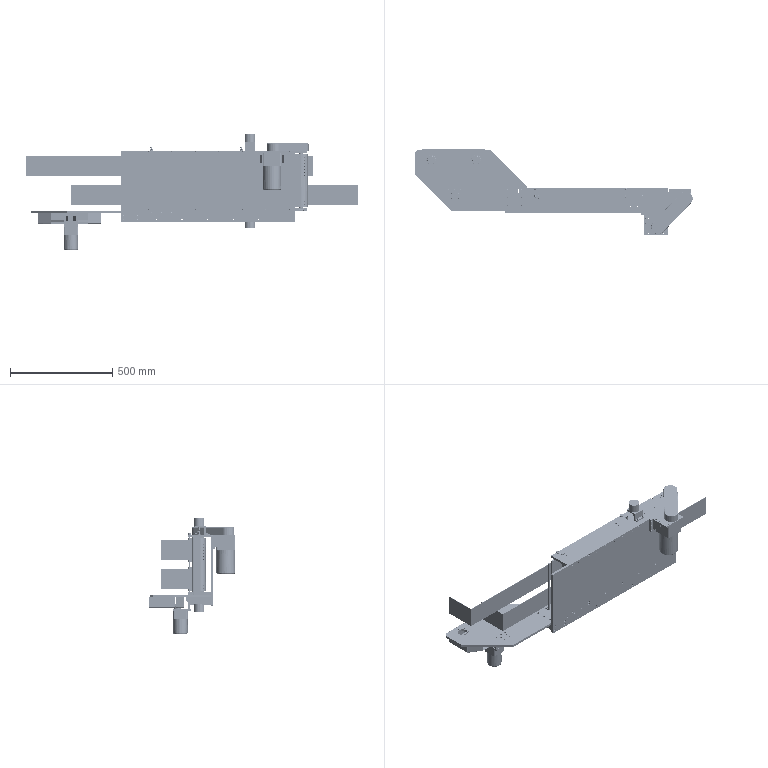Assembly | SolidWorks | mm | 75 component files | 75 solids | 4321 faces | box 1622 x 419.25 x 568 mm | volume 14757851 mm3 | cylinder 2735 | plane 960 | cone 372 | spline 244 | torus 10 | commonest cylinder face diameters 3 x1344 5 x136 4.2 x118 8 x106 5.08 x100 5.5 x93 11 x88 6.6 x88
Bill of materials:
LD101-02-35B15-d12 | 2 |  | Toothed sprocket-like disc with an integral cylindrical hub on one side and a keyed central bore; one radial hole through the hub wall.
LD101-02-35B15-d16 | 2 |  | Toothed sprocket-like disc with a tall cylindrical hub, a keyed bore and a radial hole in the hub.
LD101-02-5IK60Q1-C-5GN180K | 1 | SUS304 | Housing-like body: a square block with rounded corners and four corner holes, sitting on a cylindrical body, with a small off-centre shaft sticking out from a circular boss.
LD101-02-B6902zz(D15xD28x7)-2 | 4 | 60Si2Mn | Plain annular ring with flat faces and a large central bore; one face has two concentric recessed rings.
LD101-02-Chain35B-2 | 1 | 45 | Thin, closed, stadium-shaped (obround) band of constant width, rectangular in cross-section.
LD101-02-HexagonScrew-M6-2 | 4 |  | Short socket-head-cap-screw-like part: a cylindrical head with a hex socket on a plain cylindrical shank with a chamfered end.
LD101-02-HexagonScrew-M8X40-2 | 1 |  | Long socket-head-cap-screw-like part: a cylindrical head with a hex socket on a long plain cylindrical shank with a chamfered end.
LD101-02-Product-Q1-2-3 | 2 | POM (White) | Very thin L-shaped sheet or surface body: one long flat wall joined at a right angle to one short flat wall.
LD101-02-35B15-d10 | 1 |  | Toothed sprocket-like disc with an integral cylindrical hub, a small keyed bore and a radial hole in the hub.
LD101-02-3IK15Q1-C-3GN10K | 1 | SUS304 | Housing-like body: a square block with rounded corners and four corner holes over a cylindrical body, with a short plain off-centre shaft coming out of a circular boss.
LD101-02-Chain35B | 1 | 45 | Thin, closed band with a rounded-triangle outline: one long straight side and two converging sides, joined by rounded corners.
LD101-02--Q1108-1 | 1 | AL6061 | Flat rectangular plate with one large round through-hole near one end and seven smaller through-holes.
LD101-02--Q1109-1 | 1 | AL6061 | Thick rectangular plate/block with four holes through the large face and three holes drilled into one long narrow edge.
LD101-02--Q1110-1 | 2 | AL6061 | Solid block with a five-sided profile: a rectangle with one lower corner cut off by a long diagonal edge. Two holes are drilled into the flat top face.
LD101-02--Q1001-Q1-2 | 1 | AL6061 | Thin rectangular plate with six small holes in two columns of three, near the short ends. Its edges are beveled.
LD101-02--Q1004-Q1-2 | 2 | 45 | Long, slender cylinder with a bore along its axis, open at at least one end (tube or bored rod).
LD101-02--Q1005-Q1-2 | 2 | AL6061 | Long rectangular bar with two holes drilled into one end face.
LD101-02--Q1006-Q1-2 | 1 | 45 | Thin rectangular plate with fourteen parallel slots in two groups of seven, separated by a solid band. It has four corner holes, small V-notches at mid-height on the side edges, and beveled edges.
LD101-02--Q1011-Q1-2 | 8 | 45 | Roughly square, block-like solid with one large round through hole placed off-center. Two adjacent corners are chamfered.
LD101-02--Q1012-Q1-2 | 1 | AL6061 | Thin flat plate with an irregular outline: a long diagonal edge, a step down to a narrower rectangular extension, and a U-shaped slot open to an edge. It has two large round holes, each ringed by six small holes, plus many small holes and a short slot.
LD101-02--Q1014-Q1-2 | 1 | AL6061 | Thin, plain rectangular plate with three small holes drilled into one long edge.
LD101-02--Q1016-Q1-2 | 1 | 45 | Turned (rotationally symmetric) part: two large cylinder sections of equal diameter separated by a narrow groove, with stepped shaft ends of smaller diameter at both ends.
LD101-02--Q1017-Q1-2 | 1 | POM (White) | Thin-walled, open-ended tube with an obround (stadium-shaped) cross-section, perforated with a regular grid of small round holes in two bands separated by a solid band.
LD101-02--Q1020-Q1-2 | 1 | 45 | Long, slender, solid cylindrical rod with plain flat ends.
LD101-02--Q1024-Q1-2 | 1 | 45 | Solid of revolution: a long cylindrical body split by a narrow, shallow circumferential groove near mid-length, with small stepped shaft journals sticking out from both end faces.
LD101-02--Q1025-Q1-2 | 1 | 45 | Flat L-shaped (also readable as T-shaped) plate with one large round through hole in the main body, a chamfered corner, a long rounded-end slot running through the length of one arm, and small holes drilled into the side edges.
LD101-02--Q1026-Q1-2 | 1 | 45 | Flat L-shaped (also readable as T-shaped) plate, the same outline as unnamed part, but the large hole is stepped (counterbored) and one edge hole is larger. It also has a long rounded-end slot in one arm and chamfered corners.
LD101-02--Q1030-Q1-2 | 1 | AL6061 | Thin, large rectangular plate with slightly rounded corners and many small through holes, mostly in rows near the two long edges, plus a cluster of holes near one end.
LD101-02--Q1033-Q1-2 | 2 | AL6061 | Slender rectangular bar with two blind holes drilled into one end face. No other features are visible on the long faces.
LD101-02--Q1036-Q1-2 | 2 | AL6061 | Block with a stepped (L-shaped) cross-section: a thicker top flange overhangs a deeper web along its full length. Two round holes pass through the top flange.
LD101-02--Q1037-Q1-2 | 2 | AL6061 | Long rectangular bar whose height tapers along most of its length: one edge slopes from a full-height end to a shallower end. Three holes are in the top face and two holes are in the full-height end face.
LD101-02--Q1042-Q1-2 | 1 | AL6061 | Rectangular flat plate with one large off-center round through hole and eight smaller through holes near the perimeter, in two sizes.
LD101-02--Q1043-Q1-2 | 1 | AL6061 | Thick rectangular plate with 13 round through holes: three larger holes along each short edge, two medium holes inboard at each end, and three small holes in a row along one long edge.
LD101-02--Q1051-Q1-2 | 1 | AL6061 | Long, narrow flat plate with a stepped reduced-width end, two small U-shaped notches on one long edge, scattered small holes, one larger round hole, and a row of small holes along one long edge face.
LD101-02--Q1057-Q1-2 | 2 | AL6061 | Thick, nearly square plate with two chamfered corners on one edge, a large circular through bore, and five smaller round through holes around it.
LD101-02--Q1068-Q1-2 | 1 | AL6061 | Long, narrow flat plate with the same outline as unnamed part (stepped end, two edge notches, edge-face holes). It has extra small holes near one end and a second larger round hole, giving two larger through holes in total.
LD101-02--Q1069-Q1-2 | 2 | Nylon1010 | Thin flat rectangular plate or strip, long and narrow, with no visible holes or cutouts.
LD101-02--Q1070-Q1-2 | 2 | AL6061 | Thick plate-like block with a gusset-like profile: a short vertical edge at one side, then a long 45-degree-looking diagonal cut down to the opposite side. Two holes are drilled into one long flat narrow face.
LD101-02--Q1071-Q1-2 | 1 | SUS304 | Flat bar with a rounded-end (obround) outline, constant thickness and small edge rounds or chamfers. The shape resembles a rounded-end key.
LD101-02--Q1072-Q1-2 | 1 | SUS304 | Sheet-metal tray or cover: a flat base with an angled cut at each front corner and a U-shaped slot with a rounded end cut in from the front edge. Upturned flanges run along the back and sides, and partial flanges sit at the front. The back flange is taller and has four evenly spaced holes in a row.
LD101-02--Q1107-2 | 4 | 45 | Short thick-walled cylindrical ring or collar with a central through bore, chamfered outer edges and radial holes through the outer wall.
LD101-02-RotaryEncoder-0002-2 | 2 | AL6061 | Stepped cylindrical body: a large main cylinder, a smaller coaxial pilot boss on top and a slender cylindrical shaft sticking up from the center. The top face has three small holes spaced around the boss. The bottom face has a small circular feature at the center and three small recesses spaced around it.
LD101-02-WFSP8-0.8-10-2 | 4 |  | Shape like an extension spring: the coil is shown as a solid hollow cylindrical tube, with a round wire loop or hook at each end, and the two loops are turned relative to each other.
Mates:
1. coincident | LD101-02--Q1051-Q1-2-1 face at (-400.29, -129.897, 281.257) dir (0, 1, 0) | LD101-02--Q1068-Q1-2-2 face at (-400.29, -129.897, -0.7433) dir (0, 1, 0)
2. coincident | LD101-02--Q1051-Q1-2-1 face at (-400.29, -129.897, 281.257) dir (-1, 0, 0) | LD101-02--Q1068-Q1-2-2 face at (-400.29, -129.897, -0.7433) dir (-1, 0, 0)
3. coincident | LD101-02--Q1001-Q1-2-1 face at (-420.29, -148.897, 11.257) dir (0, 0, -1) | LD101-02--Q1068-Q1-2-2 face at (-30.29, -184.897, 11.257) dir (0, 0, 1)
4. distance | LD101-02--Q1001-Q1-2-1 face at (-420.29, -148.897, 281.257) dir (-1, 0, 0) | LD101-02--Q1068-Q1-2-2 face at (-400.29, -129.897, -0.7433) dir (-1, 0, 0)
5. coincident | LD101-02--Q1001-Q1-2-1 face at (-420.29, -148.897, 281.257) dir (0, 0, 1) | LD101-02--Q1051-Q1-2-1 face at (-30.29, -184.897, 281.257) dir (0, 0, -1)
6. distance | LD101-02--Q1001-Q1-2-1 face at (-160.29, -148.897, 146.257) dir (0, 1, 0) | LD101-02--Q1068-Q1-2-2 face at (-400.29, -129.897, -0.7433) dir (0, 1, 0)
7. concentric | LD101-02--Q1004-Q1-2-1 face at (-360.29, -135.897, 303.757) dir (0, 0, -1) r 4 | LD101-02--Q1011-Q1-2-1 face at (-360.29, -135.897, 155.257) dir (0, 0, 1) r 4
8. width | LD101-02--Q1004-Q1-2-1 face at (-360.29, -135.897, 303.757) dir (0, 0, 1) | LD101-02--Q1004-Q1-2-1 face at (-360.29, -135.897, -11.243) dir (0, 0, -1) | LD101-02--Q1068-Q1-2-2 face at (-30.29, -184.897, -0.7433) dir (0, 0, -1) | LD101-02--Q1051-Q1-2-1 face at (-30.29, -184.897, 293.257) dir (0, 0, 1)
9. concentric | LD101-02--Q1004-Q1-2-1 face at (-360.29, -135.897, 303.757) dir (0, 0, -1) r 4 | LD101-02--Q1011-Q1-2-2 face at (-360.29, -135.897, 125.257) dir (0, 0, 1) r 4
10. concentric | LD101-02--Q1051-Q1-2-1 face at (-360.29, -135.897, 281.257) dir (0, 0, 1) r 4.1 | LD101-02--Q1004-Q1-2-1 face at (-360.29, -135.897, 303.757) dir (0, 0, -1) r 4
11. coincident | LD101-02--Q1011-Q1-2-1 face at (-370.29, -129.897, 167.257) dir (0, 1, 0) | LD101-02--Q1011-Q1-2-2 face at (-370.29, -129.897, 137.257) dir (0, 1, 0)
12. concentric | LD101-02--Q1004-Q1-2-2 face at (79.71, -135.897, -11.243) dir (0, 0, 1) r 4 | LD101-02--Q1011-Q1-2-3 face at (79.71, -135.897, 139.257) dir (0, 0, -1) r 4
13. concentric | LD101-02--Q1004-Q1-2-2 face at (79.71, -135.897, -11.243) dir (0, 0, 1) r 4 | LD101-02--Q1011-Q1-2-4 face at (79.71, -135.897, 169.257) dir (0, 0, -1) r 4
14. concentric | LD101-02--Q1051-Q1-2-1 face at (79.71, -135.897, 281.257) dir (0, 0, 1) r 4.1 | LD101-02--Q1004-Q1-2-2 face at (79.71, -135.897, -11.243) dir (0, 0, 1) r 4
15. coincident | LD101-02--Q1004-Q1-2-1 face at (-360.29, -135.897, 303.757) dir (0, 0, 1) | LD101-02--Q1004-Q1-2-2 face at (79.71, -135.897, 303.757) dir (0, 0, 1)
16. coincident | LD101-02--Q1011-Q1-2-1 face at (-360.29, -139.397, 167.257) dir (0, 0, 1) | LD101-02--Q1011-Q1-2-4 face at (79.71, -139.397, 167.257) dir (0, 0, 1)
17. coincident | LD101-02--Q1011-Q1-2-2 face at (-360.29, -139.397, 137.257) dir (0, 0, 1) | LD101-02--Q1011-Q1-2-3 face at (79.71, -139.397, 137.257) dir (0, 0, 1)
18. coincident | LD101-02--Q1011-Q1-2-3 face at (89.71, -129.897, 127.257) dir (0, 1, 0) | LD101-02--Q1011-Q1-2-4 face at (89.71, -129.897, 157.257) dir (0, 1, 0)
19. concentric | LD101-02-WFSP8-0.8-10-2-1 sketch segment at (-360.29, -175.897, 299.257) dir (0, 0, 1) r 3.2 | LD101-02-HexagonScrew-M6-2-1 face at (-360.29, -175.897, 301.563) dir (0, 0, -1) r 3
20. concentric | LD101-02-WFSP8-0.8-10-2-4 sketch segment at (79.71, -175.897, 299.257) dir (0, 0, 1) r 3.2 | LD101-02-HexagonScrew-M6-2-4 face at (79.71, -175.897, 301.563) dir (0, 0, -1) r 3
21. parallel | LD101-02--Q1051-Q1-2-1 face at (339.71, -129.897, 281.257) dir (1, 0, 0) | LD101-02-WFSP8-0.8-10-2-4 plane at (79.71, -179.097, 299.257) dir (-1, 0, 0)
22. concentric | LD101-02--Q1004-Q1-2-1 face at (-360.29, -135.897, 303.757) dir (0, 0, -1) r 4 | LD101-02--Q1107-2-1 face at (-360.29, -135.897, 299.257) dir (0, 0, -1) r 4
23. coincident | LD101-02--Q1051-Q1-2-1 face at (-30.29, -184.897, 293.257) dir (0, 0, 1) | LD101-02--Q1107-2-1 face at (-360.29, -135.897, 293.257) dir (0, 0, -1)
24. coincident | LD101-02--Q1107-2-1 face at (-360.29, -135.897, 299.257) dir (0, 0, 1) | LD101-02--Q1107-2-5 face at (79.71, -135.897, 299.257) dir (0, 0, 1)
25. concentric | LD101-02--Q1004-Q1-2-2 face at (79.71, -135.897, -11.243) dir (0, 0, 1) r 4 | LD101-02--Q1107-2-5 face at (79.71, -135.897, 299.257) dir (0, 0, -1) r 4
26. width | LD101-02--Q1051-Q1-2-1 face at (-30.29, -184.897, 281.257) dir (0, 0, -1) | LD101-02--Q1068-Q1-2-2 face at (-30.29, -184.897, 11.257) dir (0, 0, 1) | LD101-02--Q1016-Q1-2-1 face at (121.71, -181.897, 16.257) dir (0, 0, -1) | LD101-02--Q1016-Q1-2-1 face at (121.71, -181.897, 276.257) dir (0, 0, 1)
27. concentric | LD101-02--Q1016-Q1-2-1 face at (121.71, -181.897, -3.743) dir (0, 0, 1) r 7.5 | LD101-02--Q1017-Q1-2-1 face at (121.71, -181.897, 276.257) dir (0, 0, -1) r 30
28. coincident | LD101-02--Q1016-Q1-2-1 face at (121.71, -181.897, 276.257) dir (0, 0, 1) | LD101-02--Q1017-Q1-2-1 face at (121.71, -181.897, 276.257) dir (0, 0, 1)
29. concentric | LD101-02--Q1016-Q1-2-1 face at (121.71, -181.897, 296.257) dir (0, 0, -1) r 7.5 | LD101-02-B6902zz(D15xD28x7)-2-1 face at (121.71, -181.897, 289.757) dir (0, 0, 1) r 7.5
30. coincident | LD101-02--Q1016-Q1-2-1 face at (121.71, -181.897, 286.257) dir (0, 0, 1) | LD101-02-B6902zz(D15xD28x7)-2-1 face at (117.578, -174.412, 286.257) dir (0, 0, -1)
31. concentric | LD101-02--Q1016-Q1-2-1 face at (121.71, -181.897, -3.743) dir (0, 0, 1) r 7.5 | LD101-02-B6902zz(D15xD28x7)-2-2 face at (121.71, -181.897, 2.757) dir (0, 0, 1) r 14
32. coincident | LD101-02--Q1016-Q1-2-1 face at (121.71, -181.897, 6.257) dir (0, 0, -1) | LD101-02-B6902zz(D15xD28x7)-2-2 face at (121.71, -173.347, 6.257) dir (0, 0, 1)
33. concentric | LD101-02--Q1017-Q1-2-1 face at (371.71, -181.897, 276.257) dir (0, 0, -1) r 30 | LD101-02--Q1024-Q1-2-1 face at (371.71, -181.897, 291.257) dir (0, 0, -1) r 7.5
34. concentric | LD101-02--Q1024-Q1-2-1 face at (371.71, -181.897, 291.257) dir (0, 0, -1) r 7.5 | LD101-02--Q1025-Q1-2-1 face at (371.71, -181.897, 288.257) dir (0, 0, -1) r 14
35. coincident | LD101-02--Q1024-Q1-2-1 face at (371.71, -181.897, 281.257) dir (0, 0, 1) | LD101-02--Q1025-Q1-2-1 face at (346.71, -132.897, 281.257) dir (0, 0, -1)
36. concentric | LD101-02--Q1024-Q1-2-1 face at (371.71, -181.897, 316.257) dir (0, 0, 1) r 6 | LD101-02--Q1026-Q1-2-1 face at (371.71, -181.897, 4.257) dir (0, 0, 1) r 14
37. coincident | LD101-02--Q1024-Q1-2-1 face at (371.71, -181.897, 11.257) dir (0, 0, -1) | LD101-02--Q1026-Q1-2-1 face at (346.71, -132.897, 11.257) dir (0, 0, 1)
38. coincident | LD101-02--Q1017-Q1-2-1 face at (121.71, -181.897, 276.257) dir (0, 0, 1) | LD101-02--Q1024-Q1-2-1 face at (371.71, -181.897, 276.257) dir (0, 0, 1)
39. coincident | LD101-02--Q1025-Q1-2-1 face at (401.71, -132.897, 293.257) dir (0, 1, 0) | LD101-02--Q1026-Q1-2-1 face at (401.71, -132.897, 11.257) dir (0, 1, 0)
40. parallel | LD101-02--Q1051-Q1-2-1 face at (-400.29, -129.897, 281.257) dir (0, 1, 0) | LD101-02--Q1025-Q1-2-1 face at (401.71, -132.897, 293.257) dir (0, 1, 0)
41. width | LD101-02--Q1068-Q1-2-2 face at (-30.29, -184.897, 11.257) dir (0, 0, 1) | LD101-02--Q1051-Q1-2-1 face at (-30.29, -184.897, 281.257) dir (0, 0, -1) | LD101-02--Q1069-Q1-2-2 face at (-370.29, -153.897, 279.257) dir (0, 0, 1) | LD101-02--Q1069-Q1-2-2 face at (-370.29, -153.897, 13.257) dir (0, 0, -1)
42. parallel | LD101-02--Q1051-Q1-2-1 face at (-400.29, -129.897, 281.257) dir (0, 1, 0) | LD101-02--Q1011-Q1-2-1 face at (-370.29, -129.897, 167.257) dir (0, 1, 0)
43. coincident | LD101-02--Q1069-Q1-2-2 face at (-370.29, -153.897, 13.257) dir (1, 0, 0) | LD101-02--Q1011-Q1-2-2 face at (-370.29, -148.897, 137.257) dir (-1, 0, 0)
44. width | LD101-02--Q1051-Q1-2-1 face at (-30.29, -184.897, 281.257) dir (0, 0, -1) | LD101-02--Q1068-Q1-2-2 face at (-30.29, -184.897, 11.257) dir (0, 0, 1) | LD101-02--Q1069-Q1-2-3 face at (69.71, -153.897, 279.257) dir (0, 0, 1) | LD101-02--Q1069-Q1-2-3 face at (69.71, -153.897, 13.257) dir (0, 0, -1)
45. coincident | LD101-02--Q1011-Q1-2-4 face at (69.71, -148.897, 157.257) dir (-1, 0, 0) | LD101-02--Q1069-Q1-2-3 face at (69.71, -153.897, 13.257) dir (1, 0, 0)
46. parallel | LD101-02--Q1051-Q1-2-1 face at (-400.29, -129.897, 281.257) dir (0, 1, 0) | LD101-02--Q1017-Q1-2-1 face at (121.71, -148.897, 276.257) dir (0, 1, 0)
47. concentric | LD101-02-HexagonScrew-M6-2-4 face at (79.71, -175.897, 301.563) dir (0, 0, -1) r 3 | LD101-02--Q1051-Q1-2-1 face at (79.71, -175.897, 293.257) dir (0, 0, 1) r 3
48. distance | LD101-02-HexagonScrew-M6-2-4 face at (79.71, -175.897, 285.257) dir (0, 0, -1) | LD101-02--Q1051-Q1-2-1 face at (-30.29, -184.897, 293.257) dir (0, 0, 1)
49. coincident | LD101-02--Q1051-Q1-2-1 face at (-400.29, -239.897, 281.257) dir (0, -1, 0) | LD101-02--Q1030-Q1-2-1 face at (-85.29, -239.897, 118.257) dir (0, 1, 0)
50. coincident | LD101-02--Q1068-Q1-2-2 face at (-30.29, -184.897, 11.257) dir (0, 0, 1) | LD101-02--Q1014-Q1-2-1 face at (244.21, -200.897, 11.257) dir (0, 0, -1)
51. coincident | LD101-02--Q1014-Q1-2-1 face at (159.21, -196.897, 281.257) dir (0, 1, 0) | LD101-02--Q1005-Q1-2-1 face at (164.21, -196.897, 146.257) dir (0, -1, 0)
52. coincident | LD101-02--Q1068-Q1-2-2 face at (-30.29, -184.897, 11.257) dir (0, 0, 1) | LD101-02--Q1005-Q1-2-1 face at (160.21, -196.897, 11.257) dir (0, 0, -1)
53. distance | LD101-02--Q1014-Q1-2-1 face at (159.21, -204.897, 281.257) dir (-1, 0, 0) | LD101-02--Q1005-Q1-2-1 face at (160.21, -196.897, 281.257) dir (-1, 0, 0)
54. coincident | LD101-02--Q1005-Q1-2-1 face at (160.21, -196.897, 281.257) dir (0, 0, 1) | LD101-02--Q1005-Q1-2-2 face at (320.21, -196.897, 281.257) dir (0, 0, 1)
55. coincident | LD101-02--Q1005-Q1-2-1 face at (164.21, -160.897, 146.257) dir (0, 1, 0) | LD101-02--Q1005-Q1-2-2 face at (324.21, -160.897, 146.257) dir (0, 1, 0)
56. distance | LD101-02--Q1005-Q1-2-2 face at (328.21, -196.897, 281.257) dir (1, 0, 0) | LD101-02--Q1014-Q1-2-1 face at (329.21, -204.897, 281.257) dir (1, 0, 0)
57. coincident | LD101-02--Q1005-Q1-2-1 face at (164.21, -160.897, 146.257) dir (0, 1, 0) | LD101-02--Q1006-Q1-2-1 face at (154.21, -160.897, 281.257) dir (0, -1, 0)
58. coincident | LD101-02--Q1005-Q1-2-1 face at (160.21, -196.897, 281.257) dir (0, 0, 1) | LD101-02--Q1006-Q1-2-1 face at (244.21, -156.897, 281.257) dir (0, 0, 1)
59. width | LD101-02--Q1006-Q1-2-1 face at (154.21, -160.897, 281.257) dir (-1, 0, 0) | LD101-02--Q1006-Q1-2-1 face at (334.21, -160.897, 281.257) dir (1, 0, 0) | LD101-02--Q1005-Q1-2-2 face at (328.21, -196.897, 281.257) dir (1, 0, 0) | LD101-02--Q1005-Q1-2-1 face at (160.21, -196.897, 281.257) dir (-1, 0, 0)
60. coincident | LD101-02--Q1068-Q1-2-2 face at (-30.29, -184.897, -0.7433) dir (0, 0, -1) | LD101-02--Q1012-Q1-2-5 face at (-600.29, -89.897, -0.7433) dir (0, 0, 1)
61. coincident | LD101-02--Q1030-Q1-2-1 face at (-85.29, -239.897, 118.257) dir (0, 1, 0) | LD101-02--Q1012-Q1-2-5 face at (-950.29, -239.897, -12.743) dir (0, -1, 0)
62. distance | LD101-02--Q1012-Q1-2-5 face at (-250.29, 60.103, -12.743) dir (1, 0, 0) | LD101-02--Q1068-Q1-2-2 face at (-400.29, -129.897, -0.7433) dir (-1, 0, 0)
63. coincident | LD101-02--Q1051-Q1-2-1 face at (339.71, -129.897, 281.257) dir (1, 0, 0) | LD101-02--Q1030-Q1-2-1 face at (339.71, -239.897, 293.257) dir (1, 0, 0)
64. coincident | LD101-02--Q1020-Q1-2-1 face at (-440.29, -154.897, -0.7433) dir (0, 0, -1) | LD101-02--Q1012-Q1-2-5 face at (-600.29, -89.897, -0.7433) dir (0, 0, 1)
65. concentric | LD101-02--Q1026-Q1-2-1 face at (361.71, -212.897, 5.257) dir (1, 0, 0) r 4 | LD101-02-HexagonScrew-M8X40-2-2 face at (375.094, -212.897, 5.257) dir (-1, 0, 0) r 4
66. coincident | LD101-02--Q1068-Q1-2-2 face at (339.71, -129.897, -0.7433) dir (1, 0, 0) | LD101-02-HexagonScrew-M8X40-2-2 face at (339.71, -212.897, 5.257) dir (-1, 0, 0)
67. coincident | LD101-02--Q1001-Q1-2-1 face at (-160.29, -156.897, 146.257) dir (0, -1, 0) | LD101-02--Q1033-Q1-2-1 face at (-350.29, -156.897, 11.257) dir (0, 1, 0)
68. width | LD101-02--Q1051-Q1-2-1 face at (-30.29, -184.897, 281.257) dir (0, 0, -1) | LD101-02--Q1068-Q1-2-2 face at (-30.29, -184.897, 11.257) dir (0, 0, 1) | LD101-02--Q1033-Q1-2-1 face at (-350.29, -186.897, 281.257) dir (0, 0, 1) | LD101-02--Q1033-Q1-2-1 face at (-350.29, -186.897, 11.257) dir (0, 0, -1)
69. coincident | LD101-02--Q1033-Q1-2-1 face at (-350.29, -186.897, 281.257) dir (0, 0, 1) | LD101-02--Q1033-Q1-2-2 face at (9.71, -186.897, 281.257) dir (0, 0, 1)
70. coincident | LD101-02--Q1033-Q1-2-1 face at (-350.29, -186.897, 11.257) dir (0, -1, 0) | LD101-02--Q1033-Q1-2-2 face at (9.71, -186.897, 11.257) dir (0, -1, 0)
71. distance | LD101-02--Q1033-Q1-2-1 face at (-350.29, -171.897, 146.257) dir (-1, 0, 0) | LD101-02--Q1068-Q1-2-2 face at (-400.29, -129.897, -0.7433) dir (-1, 0, 0)
72. coincident | LD101-02--Q1025-Q1-2-1 face at (371.71, -181.897, 288.257) dir (0, 0, -1) | LD101-02-B6902zz(D15xD28x7)-2-3 face at (371.71, -173.347, 288.257) dir (0, 0, 1)
73. concentric | LD101-02--Q1025-Q1-2-1 face at (371.71, -181.897, 288.257) dir (0, 0, -1) r 14 | LD101-02-B6902zz(D15xD28x7)-2-3 face at (371.71, -181.897, 284.757) dir (0, 0, 1) r 7.5
74. concentric | LD101-02--Q1026-Q1-2-1 face at (371.71, -181.897, 4.257) dir (0, 0, 1) r 14 | LD101-02-B6902zz(D15xD28x7)-2-4 face at (371.71, -181.897, 7.757) dir (0, 0, 1) r 7.5
75. coincident | LD101-02--Q1026-Q1-2-1 face at (371.71, -181.897, 4.257) dir (0, 0, 1) | LD101-02-B6902zz(D15xD28x7)-2-4 face at (371.71, -173.347, 4.257) dir (0, 0, -1)
76. coincident | LD101-02--Q1030-Q1-2-1 face at (-85.29, -239.897, 118.257) dir (0, 1, 0) | LD101-02--Q1037-Q1-2-1 face at (-488.29, -239.897, -12.743) dir (0, -1, 0)
77. coincident | LD101-02--Q1012-Q1-2-5 face at (-600.29, -89.897, -12.743) dir (0, 0, -1) | LD101-02--Q1037-Q1-2-1 face at (-488.29, -119.897, -12.743) dir (0, 0, 1)
78. distance | LD101-02--Q1037-Q1-2-1 face at (-500.29, -239.897, -12.743) dir (-1, 0, 0) | LD101-02--Q1030-Q1-2-1 face at (-510.29, -239.897, 293.257) dir (-1, 0, 0)
79. concentric | LD101-02--Q1068-Q1-2-2 face at (121.71, -181.897, 6.257) dir (0, 0, -1) r 14 | LD101-02--Q1016-Q1-2-1 face at (121.71, -181.897, -18.743) dir (0, 0, 1) r 4
80. coincident | LD101-02--Q1042-Q1-2-1 face at (170.211, -261.897, 293.257) dir (0, 1, 0) | LD101-02--Q1043-Q1-2-1 face at (229.211, -261.897, 258.257) dir (0, -1, 0)
81. coincident | LD101-02--Q1036-Q1-2-1 face at (146.71, -224.897, -35.743) dir (0, 0, -1) | LD101-02--Q1057-Q1-2-1 face at (121.71, -185.897, -35.743) dir (0, 0, 1)
82. concentric | LD101-02--Q1036-Q1-2-1 face at (139.71, -210.897, -35.743) dir (0, 0, -1) r 1.65 | LD101-02--Q1057-Q1-2-1 face at (139.71, -210.897, -43.743) dir (0, 0, -1) r 4
83. concentric | LD101-02--Q1036-Q1-2-1 face at (103.71, -210.897, -35.743) dir (0, 0, -1) r 1.65 | LD101-02--Q1057-Q1-2-1 face at (103.71, -210.897, -43.743) dir (0, 0, -1) r 4
84. concentric | LD101-02-RotaryEncoder-0002-2-1 face at (121.71, -181.897, -38.743) dir (0, 0, -1) r 15 | LD101-02--Q1057-Q1-2-1 face at (121.71, -181.897, -43.743) dir (0, 0, 1) r 15.05
85. coincident | LD101-02-RotaryEncoder-0002-2-1 face at (121.71, -181.897, -43.743) dir (0, 0, 1) | LD101-02--Q1057-Q1-2-1 face at (121.71, -185.897, -43.743) dir (0, 0, -1)
86. distance | LD101-02--Q1006-Q1-2-1 face at (154.21, -152.897, 281.257) dir (0, 1, 0) | LD101-02--Q1017-Q1-2-1 face at (121.71, -151.897, 276.257) dir (0, -1, 0)
87. distance | LD101-02--Q1014-Q1-2-1 face at (329.21, -204.897, 281.257) dir (1, 0, 0) | LD101-02--Q1068-Q1-2-2 face at (339.71, -129.897, -0.7433) dir (1, 0, 0)
88. distance | LD101-02--Q1033-Q1-2-1 face at (-340.29, -171.897, 146.257) dir (1, 0, 0) | LD101-02--Q1033-Q1-2-2 face at (9.71, -171.897, 146.257) dir (-1, 0, 0)
89. coincident | LD101-02-Product-Q1-2-3-1 face at (-750.29, -146.897, 127.257) dir (0, 1, 0) | LD101-02-Product-Q1-2-3-2 face at (-970.29, -146.897, 267.257) dir (0, 1, 0)
90. concentric | LD101-02--Q1016-Q1-2-1 face at (121.71, -181.897, -18.743) dir (0, 0, 1) r 4 | LD101-02-RotaryEncoder-0002-2-1 face at (121.71, -181.897, -23.743) dir (0, 0, -1) r 4
91. coincident | LD101-02--Q1068-Q1-2-2 face at (-30.29, -184.897, -0.7433) dir (0, 0, -1) | LD101-02--Q1036-Q1-2-1 face at (146.71, -224.897, -0.7433) dir (0, 0, 1)
92. parallel | LD101-02--Q1068-Q1-2-2 face at (-400.29, -129.897, -0.7433) dir (0, 1, 0) | LD101-02--Q1057-Q1-2-1 face at (147.71, -155.897, -35.743) dir (0, 1, 0)
93. concentric | LD101-02--Q1057-Q1-2-2 face at (121.71, -181.897, 336.257) dir (0, 0, -1) r 15.05 | LD101-02-RotaryEncoder-0002-2-2 face at (121.71, -181.897, 316.257) dir (0, 0, 1) r 4
94. coincident | LD101-02--Q1057-Q1-2-2 face at (121.71, -185.897, 336.257) dir (0, 0, 1) | LD101-02-RotaryEncoder-0002-2-2 face at (121.71, -181.897, 336.257) dir (0, 0, -1)
95. concentric | LD101-02--Q1036-Q1-2-2 face at (103.71, -210.897, 328.257) dir (0, 0, 1) r 1.65 | LD101-02--Q1057-Q1-2-2 face at (103.71, -210.897, 336.257) dir (0, 0, 1) r 4
96. coincident | LD101-02--Q1036-Q1-2-2 face at (96.71, -224.897, 328.257) dir (0, 0, 1) | LD101-02--Q1057-Q1-2-2 face at (121.71, -185.897, 328.257) dir (0, 0, -1)
97. concentric | LD101-02--Q1036-Q1-2-2 face at (139.71, -210.897, 328.257) dir (0, 0, 1) r 1.65 | LD101-02--Q1057-Q1-2-2 face at (139.71, -210.897, 336.257) dir (0, 0, 1) r 2.25
98. coincident | LD101-02--Q1051-Q1-2-1 face at (-30.29, -184.897, 293.257) dir (0, 0, 1) | LD101-02--Q1036-Q1-2-2 face at (96.71, -224.897, 293.257) dir (0, 0, -1)
99. concentric | LD101-02--Q1016-Q1-2-1 face at (121.71, -181.897, 296.257) dir (0, 0, -1) r 7.5 | LD101-02-RotaryEncoder-0002-2-2 face at (121.71, -181.897, 316.257) dir (0, 0, 1) r 4
100. parallel | LD101-02--Q1051-Q1-2-1 face at (-400.29, -129.897, 281.257) dir (0, 1, 0) | LD101-02--Q1057-Q1-2-2 face at (95.71, -155.897, 328.257) dir (0, 1, 0)
101. coincident | LD101-02-35B15-d16-1 face at (-650.227, 16.103, -52.743) dir (0, 0, -1) | LD101-02-35B15-d16-2 face at (-870.227, 16.103, -52.743) dir (0, 0, -1)
102. coincident | LD101-02--Q1012-Q1-2-5 face at (-600.29, -89.897, -12.743) dir (0, 0, -1) | LD101-02--Q1000-Q16-1.SLDQ1SM-1/LD101-02--Q1109-1-2 face at (-718.29, -139.897, -12.743) dir (0, 0, 1)
103. distance | LD101-02--Q1000-Q16-1.SLDQ1SM-1/LD101-02--Q1109-1-2 face at (-788.29, -139.897, -12.743) dir (-1, 0, 0) | LD101-02--Q1012-Q1-2-5 face at (-950.29, 60.103, -12.743) dir (-1, 0, 0)
104. distance | LD101-02--Q1000-Q16-1.SLDQ1SM-1/LD101-02--Q1109-1-2 face at (-753.29, -139.897, -41.743) dir (0, -1, 0) | LD101-02--Q1012-Q1-2-5 face at (-950.29, -239.897, -12.743) dir (0, -1, 0)
105. concentric | LD101-02--Q1020-Q1-2-1 face at (-440.29, -154.897, 279.257) dir (0, 0, -1) r 4 | LD101-02--Q1012-Q1-2-5 face at (-440.29, -154.897, -12.743) dir (0, 0, 1) r 2.75
106. coincident | LD101-02--Q1037-Q1-2-1 face at (-488.29, -239.897, -52.743) dir (0, 0, -1) | LD101-02--Q1037-Q1-2-2 face at (-421.29, -239.897, -52.743) dir (0, 0, -1)
107. coincident | LD101-02--Q1037-Q1-2-1 face at (-488.29, -119.897, -32.743) dir (0, 1, 0) | LD101-02--Q1037-Q1-2-2 face at (-421.29, -119.897, -32.743) dir (0, 1, 0)
108. distance | LD101-02--Q1037-Q1-2-2 face at (-433.29, -239.897, -12.743) dir (-1, 0, 0) | LD101-02--Q1030-Q1-2-1 face at (-510.29, -239.897, 293.257) dir (-1, 0, 0)
109. concentric | LD101-02--Q1004-Q1-2-1 face at (-360.29, -135.897, 303.757) dir (0, 0, -1) r 4 | LD101-02--Q1011-Q1-2-5 face at (-360.29, -135.897, 265.257) dir (0, 0, 1) r 4
110. concentric | LD101-02--Q1004-Q1-2-2 face at (79.71, -135.897, -11.243) dir (0, 0, 1) r 4 | LD101-02--Q1011-Q1-2-6 face at (79.71, -135.897, 279.257) dir (0, 0, -1) r 4
111. concentric | LD101-02--Q1004-Q1-2-2 face at (79.71, -135.897, -11.243) dir (0, 0, 1) r 4 | LD101-02--Q1011-Q1-2-7 face at (79.71, -135.897, 29.257) dir (0, 0, -1) r 4
112. coincident | LD101-02--Q1011-Q1-2-5 face at (-360.29, -139.397, 277.257) dir (0, 0, 1) | LD101-02--Q1011-Q1-2-6 face at (79.71, -139.397, 277.257) dir (0, 0, 1)
113. concentric | LD101-02--Q1004-Q1-2-1 face at (-360.29, -135.897, 303.757) dir (0, 0, -1) r 4 | LD101-02--Q1011-Q1-2-8 face at (-360.29, -135.897, 15.257) dir (0, 0, 1) r 4
114. coincident | LD101-02--Q1011-Q1-2-7 face at (79.71, -139.397, 27.257) dir (0, 0, 1) | LD101-02--Q1011-Q1-2-8 face at (-360.29, -139.397, 27.257) dir (0, 0, 1)
115. coincident | LD101-02--Q1068-Q1-2-2 face at (-400.29, -129.897, -0.7433) dir (0, 1, 0) | LD101-02--Q1011-Q1-2-8 face at (-370.29, -129.897, 27.257) dir (0, 1, 0)
116. coincident | LD101-02--Q1068-Q1-2-2 face at (-400.29, -129.897, -0.7433) dir (0, 1, 0) | LD101-02--Q1011-Q1-2-7 face at (89.71, -129.897, 17.257) dir (0, 1, 0)
117. distance | LD101-02--Q1011-Q1-2-7 face at (79.71, -139.397, 27.257) dir (0, 0, 1) | LD101-02--Q1068-Q1-2-2 face at (-30.29, -184.897, 11.257) dir (0, 0, 1)
118. distance | LD101-02--Q1011-Q1-2-3 face at (79.71, -139.397, 127.257) dir (0, 0, -1) | LD101-02--Q1011-Q1-2-7 face at (79.71, -139.397, 27.257) dir (0, 0, 1)
119. distance | LD101-02--Q1011-Q1-2-6 face at (79.71, -139.397, 267.257) dir (0, 0, -1) | LD101-02--Q1011-Q1-2-4 face at (79.71, -139.397, 167.257) dir (0, 0, 1)
120. distance | LD101-02--Q1011-Q1-2-6 face at (79.71, -139.397, 267.257) dir (0, 0, -1) | LD101-02--Q1051-Q1-2-1 face at (-30.29, -184.897, 281.257) dir (0, 0, -1)
121. coincident | LD101-02--Q1042-Q1-2-1 face at (229.211, -309.397, 283.257) dir (0, 0, -1) | LD101-02-5IK60Q1-C-5GN180K-1 face at (190.211, -350.897, 283.257) dir (0, 0, 1)
122. concentric | LD101-02--Q1042-Q1-2-1 face at (247.211, -311.897, 293.257) dir (0, 0, -1) r 17.1 | LD101-02-5IK60Q1-C-5GN180K-1 face at (247.211, -311.897, 287.257) dir (0, 0, -1) r 17
123. coincident | LD101-02--Q1042-Q1-2-1 face at (229.211, -309.397, 293.257) dir (0, 0, 1) | LD101-02--Q1043-Q1-2-1 face at (156.711, -251.897, 293.257) dir (0, 0, 1)
124. width | LD101-02--Q1042-Q1-2-1 face at (170.211, -356.897, 293.257) dir (-1, 0, 0) | LD101-02--Q1042-Q1-2-1 face at (288.211, -356.897, 293.257) dir (1, 0, 0) | LD101-02--Q1043-Q1-2-1 face at (156.711, -251.897, 293.257) dir (-1, 0, 0) | LD101-02--Q1043-Q1-2-1 face at (301.711, -251.897, 293.257) dir (1, 0, 0)
125. parallel | LD101-02--Q1042-Q1-2-1 face at (170.211, -356.897, 293.257) dir (0, -1, 0) | LD101-02-5IK60Q1-C-5GN180K-1 face at (190.211, -356.897, 216.257) dir (0, -1, 0)
126. coincident | LD101-02--Q1030-Q1-2-1 face at (-85.29, -251.897, 118.257) dir (0, -1, 0) | LD101-02--Q1043-Q1-2-1 face at (229.211, -251.897, 258.257) dir (0, 1, 0)
127. coincident | LD101-02--Q1070-Q1-2-1 face at (286.711, -261.897, 233.257) dir (0, 1, 0) | LD101-02--Q1070-Q1-2-2 face at (181.711, -261.897, 233.257) dir (0, 1, 0)
128. coincident | LD101-02--Q1070-Q1-2-1 face at (286.711, -261.897, 283.257) dir (0, 0, 1) | LD101-02--Q1070-Q1-2-2 face at (181.711, -261.897, 283.257) dir (0, 0, 1)
129. coincident | LD101-02--Q1042-Q1-2-1 face at (229.211, -309.397, 283.257) dir (0, 0, -1) | LD101-02--Q1070-Q1-2-2 face at (181.711, -261.897, 283.257) dir (0, 0, 1)
130. coincident | LD101-02--Q1043-Q1-2-1 face at (229.211, -261.897, 258.257) dir (0, -1, 0) | LD101-02--Q1070-Q1-2-2 face at (181.711, -261.897, 233.257) dir (0, 1, 0)
131. distance | LD101-02--Q1070-Q1-2-1 face at (276.711, -261.897, 283.257) dir (-1, 0, 0) | LD101-02-5IK60Q1-C-5GN180K-1 face at (274.211, -272.897, 216.257) dir (1, 0, 0)
132. distance | LD101-02--Q1070-Q1-2-2 face at (181.711, -261.897, 283.257) dir (1, 0, 0) | LD101-02-5IK60Q1-C-5GN180K-1 face at (184.211, -272.897, 216.257) dir (-1, 0, 0)
133. coincident | LD101-02-35B15-d12-1 face at (250.648, -308.265, 316.257) dir (0, 0, 1) | LD101-02-35B15-d12-2 face at (372.152, -176.917, 316.257) dir (0, 0, 1)
134. concentric | LD101-02--Q1024-Q1-2-1 face at (371.71, -181.897, 316.257) dir (0, 0, -1) r 6 | LD101-02-35B15-d12-2 face at (371.71, -181.897, 317.049) dir (0, 0, -1) r 6
135. distance | LD101-02-35B15-d12-2 face at (373.213, -164.964, 296.257) dir (0, 0, -1) | LD101-02--Q1024-Q1-2-1 face at (371.71, -181.897, 316.257) dir (0, 0, 1)
136. concentric | LD101-02-5IK60Q1-C-5GN180K-1 face at (247.211, -311.897, 315.257) dir (0, 0, -1) r 6 | LD101-02-35B15-d12-1 face at (247.211, -311.897, 316.257) dir (0, 0, -1) r 17.5
137. distance | LD101-02-5IK60Q1-C-5GN180K-1 face at (247.211, -311.897, 315.257) dir (0, 0, 1) | LD101-02-35B15-d12-1 face at (250.648, -308.265, 316.257) dir (0, 0, 1)
138. concentric | LD101-02-35B15-d12-2 face at (371.71, -181.897, 316.257) dir (0, 0, -1) r 17.5 | LD101-02-Chain35B-2-1 face at (371.71, -181.897, 320.107) dir (0, 0, -1) r 29.41
139. width | LD101-02-35B15-d12-2 face at (372.152, -176.917, 316.257) dir (0, 0, 1) | LD101-02-35B15-d12-2 face at (373.544, -161.24, 311.957) dir (0, 0, -1) | LD101-02-Chain35B-2-1 face at (371.71, -181.897, 308.107) dir (0, 0, -1) | LD101-02-Chain35B-2-1 face at (371.71, -181.897, 320.107) dir (0, 0, 1)
140. concentric | LD101-02-35B15-d12-1 face at (247.211, -311.897, 316.257) dir (0, 0, -1) r 17.5 | LD101-02-Chain35B-2-1 face at (247.211, -311.897, 320.107) dir (0, 0, -1) r 24.41
141. coincident | LD101-02--Q1051-Q1-2-1 face at (-30.29, -184.897, 293.257) dir (0, 0, 1) | LD101-02--Q1030-Q1-2-1 face at (-510.29, -239.897, 293.257) dir (0, 0, 1)
142. coincident | LD101-02--Q1042-Q1-2-1 face at (229.211, -309.397, 293.257) dir (0, 0, 1) | LD101-02--Q1071-Q1-2-1 face at (240.081, -319.935, 293.257) dir (0, 0, -1)
143. distance | LD101-02-Chain35B-2-1 face at (392.951, -202.239, 320.107) dir (0.7222, -0.6917, 0) | LD101-02--Q1071-Q1-2-1 face at (264.636, -343.452, 327.257) dir (0.7222, -0.6917, 0)
144. coincident | LD101-02--Q1012-Q1-2-5 face at (-600.29, -89.897, -0.7433) dir (0, 0, 1) | LD101-02--Q1072-Q1-2-1 face at (-607.026, 62.351, -0.7433) dir (0, 0, 1)
145. distance | LD101-02--Q1072-Q1-2-1 face at (-915.29, -22.649, -62.743) dir (-1, 0, 0) | LD101-02--Q1012-Q1-2-5 face at (-950.29, 60.103, -12.743) dir (-1, 0, 0)
146. coincident | LD101-02--Q1001-Q1-2-1 face at (-160.29, -153.897, 146.257) dir (0, 1, 0) | LD101-02--Q1069-Q1-2-2 face at (-390.29, -153.897, 146.257) dir (0, -1, 0)
147. coincident | LD101-02--Q1001-Q1-2-1 face at (-160.29, -153.897, 146.257) dir (0, 1, 0) | LD101-02--Q1069-Q1-2-3 face at (49.71, -153.897, 146.257) dir (0, -1, 0)
148. coincident | LD101-02--Q1001-Q1-2-1 face at (-160.29, -148.897, 146.257) dir (0, 1, 0) | LD101-02-Product-Q1-2-3-1 face at (-750.29, -148.897, 127.257) dir (0, -1, 0)
149. parallel | LD101-02-3IK15Q1-C-3GN10K-1 face at (-130.057, -69.171, -42.576) dir (0, 0, -1) | LD101-02--Q1000-Q16-1.SLDQ1SM plane at (0, 0, 0) dir (0, 0, 1)
150. concentric | LD101-02-3IK15Q1-C-3GN10K-1 face at (-59.057, -98.171, -22.576) dir (-1, 0, 0) r 5 | LD101-02--Q1108-1-1 face at (-91.057, -98.171, -22.576) dir (1, 0, 0) r 15.1
151. coincident | LD101-02-3IK15Q1-C-3GN10K-1 face at (-91.057, -127.171, 21.424) dir (1, 0, 0) | LD101-02--Q1108-1-1 face at (-91.057, -98.171, -0.07593) dir (-1, 0, 0)
152. parallel | LD101-02-3IK15Q1-C-3GN10K-1 face at (-130.057, -63.171, 21.424) dir (0, 1, 0) | LD101-02--Q1108-1-1 face at (-91.057, -63.171, 42.424) dir (0, 1, 0)
153. coincident | LD101-02--Q1108-1-1 face at (-81.057, -98.171, -0.07593) dir (1, 0, 0) | LD101-02--Q1109-1-2 face at (-81.057, -133.171, 41.424) dir (-1, 0, 0)
154. coincident | LD101-02--Q1108-1-1 face at (-91.057, -63.171, 42.424) dir (0, 1, 0) | LD101-02--Q1109-1-2 face at (-23.057, -63.171, 41.424) dir (0, 1, 0)
155. distance | LD101-02--Q1108-1-1 face at (-91.057, -133.171, 42.424) dir (0, 0, 1) | LD101-02--Q1109-1-2 face at (-52.057, -98.171, 41.424) dir (0, 0, 1)
156. coincident | LD101-02--Q1110-1-2 face at (-23.057, -111.171, 41.424) dir (0, 0, -1) | LD101-02--Q1109-1-2 face at (-52.057, -98.171, 41.424) dir (0, 0, 1)
157. coincident | LD101-02--Q1110-1-2 face at (-23.057, -111.171, 91.424) dir (1, 0, 0) | LD101-02--Q1109-1-2 face at (-23.057, -133.171, 41.424) dir (1, 0, 0)
158. coincident | LD101-02--Q1110-1-1 face at (-23.057, -75.171, 91.424) dir (1, 0, 0) | LD101-02--Q1110-1-2 face at (-23.057, -111.171, 91.424) dir (1, 0, 0)
159. coincident | LD101-02--Q1110-1-1 face at (-23.057, -75.171, 41.424) dir (0, 0, -1) | LD101-02--Q1109-1-2 face at (-52.057, -98.171, 41.424) dir (0, 0, 1)
160. distance | LD101-02--Q1110-1-1 face at (-23.057, -75.171, 41.424) dir (0, 1, 0) | LD101-02--Q1109-1-2 face at (-23.057, -63.171, 41.424) dir (0, 1, 0)
161. distance | LD101-02--Q1110-1-2 face at (-23.057, -121.171, 41.424) dir (0, -1, 0) | LD101-02--Q1109-1-2 face at (-23.057, -133.171, 41.424) dir (0, -1, 0)
162. concentric | LD101-02-3IK15Q1-C-3GN10K-1 face at (-59.057, -98.171, -22.576) dir (-1, 0, 0) r 5 | LD101-02-35B15-d10-1 face at (-59.057, -98.171, -22.576) dir (-1, 0, 0) r 5
163. distance | LD101-02-3IK15Q1-C-3GN10K-1 face at (-59.057, -98.171, -22.576) dir (1, 0, 0) | LD101-02-35B15-d10-1 face at (-79.057, -81.174, -22.272) dir (-1, 0, 0)
164. width | LD101-02-35B15-d10-1 face at (-63.357, -77.437, -22.206) dir (-1, 0, 0) | LD101-02-35B15-d10-1 face at (-59.057, -93.172, -22.487) dir (1, 0, 0) | LD101-02-Chain35B-1 face at (-55.207, -98.171, -22.576) dir (1, 0, 0) | LD101-02-Chain35B-1 face at (-67.207, -98.171, -22.576) dir (-1, 0, 0)
165. parallel | LD101-02--Q1108-1-1 face at (-91.057, -133.171, -42.576) dir (0, 0, -1) | LD101-02-Chain35B-1 face at (-67.207, 18.829, -138.986) dir (0, 0, -1)
166. concentric | LD101-02-35B15-d10-1 face at (-59.057, -98.171, -22.576) dir (-1, 0, 0) r 17.5 | LD101-02-Chain35B-1 face at (-67.207, -98.171, -22.576) dir (1, 0, 0) r 29.41